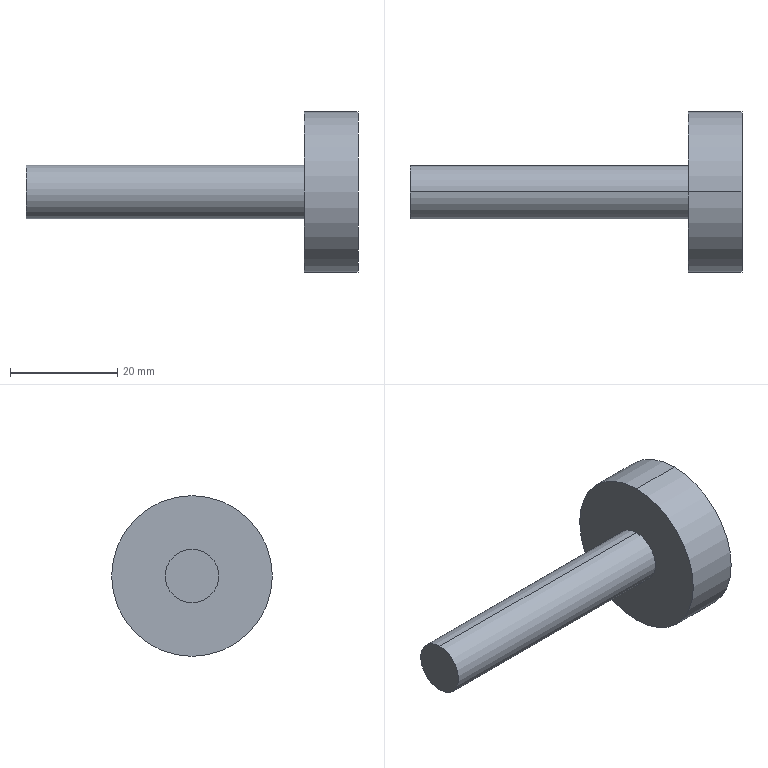Component | SolidWorks | Part3^Assembly2-1 | 1 solid | 7 faces | box 62 x 30 x 30 mm | volume 11153 mm3 | cylinder 4 | plane 3 | commonest cylinder face diameters 10 x2 30 x2
STEP:
#1=CARTESIAN_POINT('',(4.298,14.393,-35.682));
#2=VERTEX_POINT('',#1);
#3=CARTESIAN_POINT('',(4.298,14.393,-36.076));
#4=VERTEX_POINT('',#3);
#5=CARTESIAN_POINT('',(4.298,14.393,-35.879));
#6=DIRECTION('',(-1.,-0.,-0.));
#7=DIRECTION('',(0.,0.,1.));
#8=AXIS2_PLACEMENT_3D('',#5,#6,#7);
#9=CIRCLE('',#8,0.1969);
#10=EDGE_CURVE('',#2,#4,#9,.T.);
#11=ORIENTED_EDGE('',*,*,#10,.F.);
#12=CARTESIAN_POINT('',(6.346,14.393,-35.682));
#13=VERTEX_POINT('',#12);
#14=CARTESIAN_POINT('',(4.298,14.393,-35.682));
#15=DIRECTION('',(1.,0.,0.));
#16=VECTOR('',#15,39.37);
#17=LINE('',#14,#16);
#18=EDGE_CURVE('',#2,#13,#17,.T.);
#19=ORIENTED_EDGE('',*,*,#18,.T.);
#20=CARTESIAN_POINT('',(6.346,14.393,-36.076));
#21=VERTEX_POINT('',#20);
#22=CARTESIAN_POINT('',(6.346,14.393,-35.879));
#23=DIRECTION('',(-1.,-0.,-0.));
#24=DIRECTION('',(0.,0.,1.));
#25=AXIS2_PLACEMENT_3D('',#22,#23,#24);
#26=CIRCLE('',#25,0.1969);
#27=EDGE_CURVE('',#13,#21,#26,.T.);
#28=ORIENTED_EDGE('',*,*,#27,.T.);
#29=CARTESIAN_POINT('',(4.298,14.393,-36.076));
#30=DIRECTION('',(1.,0.,0.));
#31=VECTOR('',#30,39.37);
#32=LINE('',#29,#31);
#33=EDGE_CURVE('',#4,#21,#32,.T.);
#34=ORIENTED_EDGE('',*,*,#33,.F.);
#35=EDGE_LOOP('',(#11,#19,#28,#34));
#36=FACE_OUTER_BOUND('',#35,.T.);
#37=CARTESIAN_POINT('',(4.298,14.393,-35.879));
#38=DIRECTION('',(1.,0.,0.));
#39=DIRECTION('',(0.,0.,-1.));
#40=AXIS2_PLACEMENT_3D('',#37,#38,#39);
#41=CYLINDRICAL_SURFACE('',#40,0.1969);
#42=ADVANCED_FACE('',(#36),#41,.T.);
#43=CARTESIAN_POINT('',(6.739,14.393,-36.47));
#44=VERTEX_POINT('',#43);
#45=CARTESIAN_POINT('',(6.739,14.393,-35.289));
#46=VERTEX_POINT('',#45);
#47=CARTESIAN_POINT('',(6.739,14.393,-35.879));
#48=DIRECTION('',(1.,0.,0.));
#49=DIRECTION('',(0.,0.,-1.));
#50=AXIS2_PLACEMENT_3D('',#47,#48,#49);
#51=CIRCLE('',#50,0.5906);
#52=EDGE_CURVE('',#44,#46,#51,.T.);
#53=ORIENTED_EDGE('',*,*,#52,.F.);
#54=CARTESIAN_POINT('',(6.346,14.393,-36.47));
#55=VERTEX_POINT('',#54);
#56=CARTESIAN_POINT('',(6.739,14.393,-36.47));
#57=DIRECTION('',(-1.,-0.,-0.));
#58=VECTOR('',#57,39.37);
#59=LINE('',#56,#58);
#60=EDGE_CURVE('',#44,#55,#59,.T.);
#61=ORIENTED_EDGE('',*,*,#60,.T.);
#62=CARTESIAN_POINT('',(6.346,14.393,-35.289));
#63=VERTEX_POINT('',#62);
#64=CARTESIAN_POINT('',(6.346,14.393,-35.879));
#65=DIRECTION('',(1.,0.,0.));
#66=DIRECTION('',(0.,0.,-1.));
#67=AXIS2_PLACEMENT_3D('',#64,#65,#66);
#68=CIRCLE('',#67,0.5906);
#69=EDGE_CURVE('',#55,#63,#68,.T.);
#70=ORIENTED_EDGE('',*,*,#69,.T.);
#71=CARTESIAN_POINT('',(6.739,14.393,-35.289));
#72=DIRECTION('',(-1.,-0.,-0.));
#73=VECTOR('',#72,39.37);
#74=LINE('',#71,#73);
#75=EDGE_CURVE('',#46,#63,#74,.T.);
#76=ORIENTED_EDGE('',*,*,#75,.F.);
#77=EDGE_LOOP('',(#53,#61,#70,#76));
#78=FACE_OUTER_BOUND('',#77,.T.);
#79=CARTESIAN_POINT('',(6.739,14.393,-35.879));
#80=DIRECTION('',(-1.,-0.,-0.));
#81=DIRECTION('',(0.,0.,1.));
#82=AXIS2_PLACEMENT_3D('',#79,#80,#81);
#83=CYLINDRICAL_SURFACE('',#82,0.5906);
#84=ADVANCED_FACE('',(#78),#83,.T.);
#85=ORIENTED_EDGE('',*,*,#60,.F.);
#86=CARTESIAN_POINT('',(6.739,14.393,-35.879));
#87=DIRECTION('',(1.,0.,0.));
#88=DIRECTION('',(0.,0.,-1.));
#89=AXIS2_PLACEMENT_3D('',#86,#87,#88);
#90=CIRCLE('',#89,0.5906);
#91=EDGE_CURVE('',#46,#44,#90,.T.);
#92=ORIENTED_EDGE('',*,*,#91,.F.);
#93=ORIENTED_EDGE('',*,*,#75,.T.);
#94=CARTESIAN_POINT('',(6.346,14.393,-35.879));
#95=DIRECTION('',(1.,0.,0.));
#96=DIRECTION('',(0.,0.,-1.));
#97=AXIS2_PLACEMENT_3D('',#94,#95,#96);
#98=CIRCLE('',#97,0.5906);
#99=EDGE_CURVE('',#63,#55,#98,.T.);
#100=ORIENTED_EDGE('',*,*,#99,.T.);
#101=EDGE_LOOP('',(#85,#92,#93,#100));
#102=FACE_OUTER_BOUND('',#101,.T.);
#103=CARTESIAN_POINT('',(6.739,14.393,-35.879));
#104=DIRECTION('',(-1.,-0.,-0.));
#105=DIRECTION('',(0.,0.,1.));
#106=AXIS2_PLACEMENT_3D('',#103,#104,#105);
#107=CYLINDRICAL_SURFACE('',#106,0.5906);
#108=ADVANCED_FACE('',(#102),#107,.T.);
#109=ORIENTED_EDGE('',*,*,#91,.T.);
#110=ORIENTED_EDGE('',*,*,#52,.T.);
#111=EDGE_LOOP('',(#109,#110));
#112=FACE_OUTER_BOUND('',#111,.T.);
#113=CARTESIAN_POINT('',(6.739,14.393,-35.879));
#114=DIRECTION('',(1.,0.,0.));
#115=DIRECTION('',(0.,0.,-1.));
#116=AXIS2_PLACEMENT_3D('',#113,#114,#115);
#117=PLANE('',#116);
#118=ADVANCED_FACE('',(#112),#117,.T.);
#119=CARTESIAN_POINT('',(6.346,14.393,-35.879));
#120=DIRECTION('',(-1.,-0.,-0.));
#121=DIRECTION('',(0.,0.,1.));
#122=AXIS2_PLACEMENT_3D('',#119,#120,#121);
#123=CIRCLE('',#122,0.1969);
#124=EDGE_CURVE('',#21,#13,#123,.T.);
#125=ORIENTED_EDGE('',*,*,#124,.F.);
#126=ORIENTED_EDGE('',*,*,#27,.F.);
#127=EDGE_LOOP('',(#125,#126));
#128=FACE_BOUND('',#127,.T.);
#129=ORIENTED_EDGE('',*,*,#99,.F.);
#130=ORIENTED_EDGE('',*,*,#69,.F.);
#131=EDGE_LOOP('',(#129,#130));
#132=FACE_OUTER_BOUND('',#131,.T.);
#133=CARTESIAN_POINT('',(6.346,14.393,-35.879));
#134=DIRECTION('',(1.,0.,0.));
#135=DIRECTION('',(0.,0.,-1.));
#136=AXIS2_PLACEMENT_3D('',#133,#134,#135);
#137=PLANE('',#136);
#138=ADVANCED_FACE('',(#128,#132),#137,.F.);
#139=ORIENTED_EDGE('',*,*,#18,.F.);
#140=CARTESIAN_POINT('',(4.298,14.393,-35.879));
#141=DIRECTION('',(-1.,-0.,-0.));
#142=DIRECTION('',(0.,0.,1.));
#143=AXIS2_PLACEMENT_3D('',#140,#141,#142);
#144=CIRCLE('',#143,0.1969);
#145=EDGE_CURVE('',#4,#2,#144,.T.);
#146=ORIENTED_EDGE('',*,*,#145,.F.);
#147=ORIENTED_EDGE('',*,*,#33,.T.);
#148=ORIENTED_EDGE('',*,*,#124,.T.);
#149=EDGE_LOOP('',(#139,#146,#147,#148));
#150=FACE_OUTER_BOUND('',#149,.T.);
#151=CARTESIAN_POINT('',(4.298,14.393,-35.879));
#152=DIRECTION('',(1.,0.,0.));
#153=DIRECTION('',(0.,0.,-1.));
#154=AXIS2_PLACEMENT_3D('',#151,#152,#153);
#155=CYLINDRICAL_SURFACE('',#154,0.1969);
#156=ADVANCED_FACE('',(#150),#155,.T.);
#157=ORIENTED_EDGE('',*,*,#145,.T.);
#158=ORIENTED_EDGE('',*,*,#10,.T.);
#159=EDGE_LOOP('',(#157,#158));
#160=FACE_OUTER_BOUND('',#159,.T.);
#161=CARTESIAN_POINT('',(4.298,14.393,-35.879));
#162=DIRECTION('',(-1.,-0.,-0.));
#163=DIRECTION('',(-0.,-0.,1.));
#164=AXIS2_PLACEMENT_3D('',#161,#162,#163);
#165=PLANE('',#164);
#166=ADVANCED_FACE('',(#160),#165,.T.);
#167=CLOSED_SHELL('',(#42,#84,#108,#118,#138,#156,#166));
#168=MANIFOLD_SOLID_BREP('',#167);
#169=CARTESIAN_POINT('',(0.,0.,0.));
#170=DIRECTION('',(0.,0.,1.));
#171=DIRECTION('',(1.,0.,0.));
#172=AXIS2_PLACEMENT_3D('',#169,#170,#171);
#173=(LENGTH_UNIT()NAMED_UNIT(*)SI_UNIT($,.METRE.));
#174=LENGTH_MEASURE_WITH_UNIT(LENGTH_MEASURE(0.0254),#173);
#175=DIMENSIONAL_EXPONENTS(1.,0.,0.,0.,0.,0.,0.);
#176=(CONVERSION_BASED_UNIT('',#174)LENGTH_UNIT()NAMED_UNIT(#175));
#177=UNCERTAINTY_MEASURE_WITH_UNIT(LENGTH_MEASURE(0.00001),#176,'','');
#178=(NAMED_UNIT(*)PLANE_ANGLE_UNIT()SI_UNIT($,.RADIAN.));
#179=(NAMED_UNIT(*)SI_UNIT($,.STERADIAN.)SOLID_ANGLE_UNIT());
#180=(GEOMETRIC_REPRESENTATION_CONTEXT(3)GLOBAL_UNCERTAINTY_ASSIGNED_CONTEXT((#177))GLOBAL_UNIT_ASSIGNED_CONTEXT((#176,#178,#179))REPRESENTATION_CONTEXT('',''));
#181=ADVANCED_BREP_SHAPE_REPRESENTATION('',(#168,#172),#180);
#182=COLOUR_RGB('',0.7922,0.8196,0.9333);
#183=FILL_AREA_STYLE_COLOUR('',#182);
#184=FILL_AREA_STYLE('',(#183));
#185=SURFACE_STYLE_FILL_AREA(#184);
#186=SURFACE_SIDE_STYLE('',(#185));
#187=SURFACE_STYLE_USAGE(.BOTH.,#186);
#188=PRESENTATION_STYLE_ASSIGNMENT((#187));
#189=STYLED_ITEM('',(#188),#168);
#190=PRESENTATION_LAYER_ASSIGNMENT('','',(#189));
#191=(LENGTH_UNIT()NAMED_UNIT(*)SI_UNIT($,.METRE.));
#192=LENGTH_MEASURE_WITH_UNIT(LENGTH_MEASURE(0.0254),#191);
#193=DIMENSIONAL_EXPONENTS(1.,0.,0.,0.,0.,0.,0.);
#194=(CONVERSION_BASED_UNIT('',#192)LENGTH_UNIT()NAMED_UNIT(#193));
#195=UNCERTAINTY_MEASURE_WITH_UNIT(LENGTH_MEASURE(0.00001),#194,'','');
#196=(NAMED_UNIT(*)PLANE_ANGLE_UNIT()SI_UNIT($,.RADIAN.));
#197=(NAMED_UNIT(*)SI_UNIT($,.STERADIAN.)SOLID_ANGLE_UNIT());
#198=(GEOMETRIC_REPRESENTATION_CONTEXT(3)GLOBAL_UNCERTAINTY_ASSIGNED_CONTEXT((#195))GLOBAL_UNIT_ASSIGNED_CONTEXT((#194,#196,#197))REPRESENTATION_CONTEXT('',''));
#199=MECHANICAL_DESIGN_GEOMETRIC_PRESENTATION_REPRESENTATION('',(#189),#198);